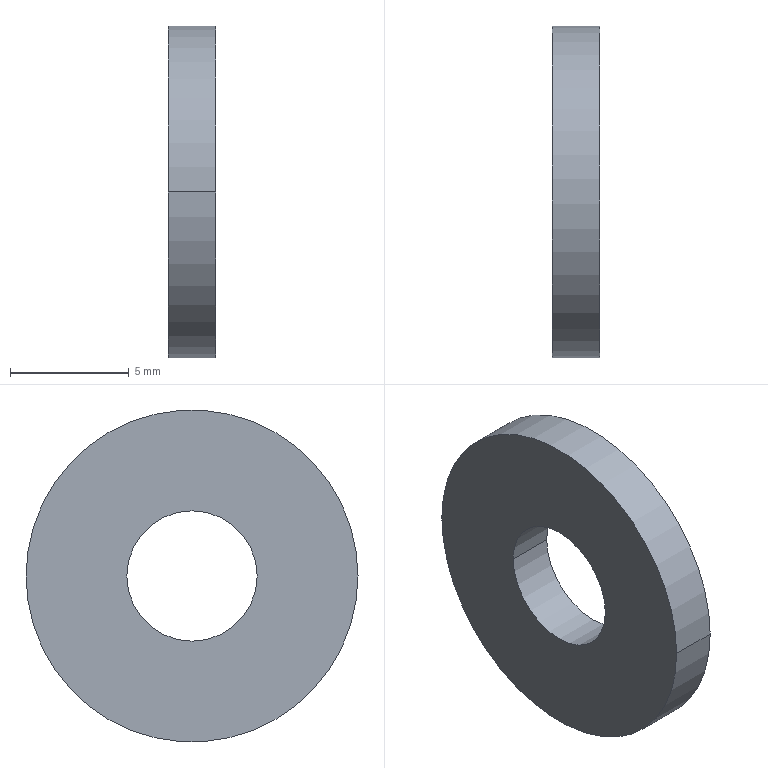Component | SolidWorks | 09HHHHHH6-1 | 1 solid | 6 faces | box 2 x 14 x 14 mm | volume 260 mm3 | cylinder 4 | plane 2 | commonest cylinder face diameters 5.5 x2 14 x2
build123d program:
from build123d import *

# Parameters (mm, degrees)
SKETCH1_R           = 7
SKETCH1_R_2         = 2.75
BOSS_EXTRUDE1_DEPTH = 2


with BuildPart() as part:
    # Sketch1 → Boss-Extrude1 (new body)
    with BuildSketch(Plane.XY):
        with Locations((302.287, -36.6)):
            Circle(SKETCH1_R)
        with Locations((302.287, -36.6)):
            Circle(SKETCH1_R_2, mode=Mode.SUBTRACT)
    extrude(amount=BOSS_EXTRUDE1_DEPTH)


solid = part.part

# Placed as in the assembly
solid = solid.moved(Location((-649.859, -249.783, 272.031), (0, 90, 0)))
STEP:
#1=COLOUR_RGB('',0.7922,0.8196,0.9333);
#2=FILL_AREA_STYLE_COLOUR('',#1);
#3=FILL_AREA_STYLE('',(#2));
#4=SURFACE_STYLE_FILL_AREA(#3);
#5=SURFACE_SIDE_STYLE('',(#4));
#6=SURFACE_STYLE_USAGE(.BOTH.,#5);
#7=PRESENTATION_STYLE_ASSIGNMENT((#6));
#8=CARTESIAN_POINT('',(-25.585,-11.167,-1.191));
#9=VERTEX_POINT('',#8);
#10=CARTESIAN_POINT('',(-25.585,-11.383,-1.191));
#11=VERTEX_POINT('',#10);
#12=CARTESIAN_POINT('',(-25.585,-11.275,-1.191));
#13=DIRECTION('',(-1.,0.,0.));
#14=DIRECTION('',(0.,-1.,0.));
#15=AXIS2_PLACEMENT_3D('',#12,#13,#14);
#16=CIRCLE('',#15,0.1083);
#17=EDGE_CURVE('',#9,#11,#16,.T.);
#18=ORIENTED_EDGE('',*,*,#17,.T.);
#19=CARTESIAN_POINT('',(-25.506,-11.383,-1.191));
#20=VERTEX_POINT('',#19);
#21=CARTESIAN_POINT('',(-25.585,-11.383,-1.191));
#22=DIRECTION('',(1.,0.,0.));
#23=VECTOR('',#22,39.37);
#24=LINE('',#21,#23);
#25=EDGE_CURVE('',#11,#20,#24,.T.);
#26=ORIENTED_EDGE('',*,*,#25,.T.);
#27=CARTESIAN_POINT('',(-25.506,-11.167,-1.191));
#28=VERTEX_POINT('',#27);
#29=CARTESIAN_POINT('',(-25.506,-11.275,-1.191));
#30=DIRECTION('',(-1.,0.,0.));
#31=DIRECTION('',(0.,-1.,0.));
#32=AXIS2_PLACEMENT_3D('',#29,#30,#31);
#33=CIRCLE('',#32,0.1083);
#34=EDGE_CURVE('',#28,#20,#33,.T.);
#35=ORIENTED_EDGE('',*,*,#34,.F.);
#36=CARTESIAN_POINT('',(-25.585,-11.167,-1.191));
#37=DIRECTION('',(1.,0.,0.));
#38=VECTOR('',#37,39.37);
#39=LINE('',#36,#38);
#40=EDGE_CURVE('',#9,#28,#39,.T.);
#41=ORIENTED_EDGE('',*,*,#40,.F.);
#42=EDGE_LOOP('',(#18,#26,#35,#41));
#43=FACE_OUTER_BOUND('',#42,.T.);
#44=CARTESIAN_POINT('',(-25.585,-11.275,-1.191));
#45=DIRECTION('',(1.,0.,0.));
#46=DIRECTION('',(0.,1.,0.));
#47=AXIS2_PLACEMENT_3D('',#44,#45,#46);
#48=CYLINDRICAL_SURFACE('',#47,0.1083);
#49=ADVANCED_FACE('',(#43),#48,.F.);
#50=CARTESIAN_POINT('',(-25.585,-11.551,-1.191));
#51=VERTEX_POINT('',#50);
#52=CARTESIAN_POINT('',(-25.585,-10.999,-1.191));
#53=VERTEX_POINT('',#52);
#54=CARTESIAN_POINT('',(-25.585,-11.275,-1.191));
#55=DIRECTION('',(-1.,0.,0.));
#56=DIRECTION('',(0.,-1.,0.));
#57=AXIS2_PLACEMENT_3D('',#54,#55,#56);
#58=CIRCLE('',#57,0.2756);
#59=EDGE_CURVE('',#51,#53,#58,.T.);
#60=ORIENTED_EDGE('',*,*,#59,.F.);
#61=CARTESIAN_POINT('',(-25.506,-11.551,-1.191));
#62=VERTEX_POINT('',#61);
#63=CARTESIAN_POINT('',(-25.585,-11.551,-1.191));
#64=DIRECTION('',(1.,0.,0.));
#65=VECTOR('',#64,39.37);
#66=LINE('',#63,#65);
#67=EDGE_CURVE('',#51,#62,#66,.T.);
#68=ORIENTED_EDGE('',*,*,#67,.T.);
#69=CARTESIAN_POINT('',(-25.506,-10.999,-1.191));
#70=VERTEX_POINT('',#69);
#71=CARTESIAN_POINT('',(-25.506,-11.275,-1.191));
#72=DIRECTION('',(-1.,0.,0.));
#73=DIRECTION('',(0.,-1.,0.));
#74=AXIS2_PLACEMENT_3D('',#71,#72,#73);
#75=CIRCLE('',#74,0.2756);
#76=EDGE_CURVE('',#62,#70,#75,.T.);
#77=ORIENTED_EDGE('',*,*,#76,.T.);
#78=CARTESIAN_POINT('',(-25.585,-10.999,-1.191));
#79=DIRECTION('',(1.,0.,0.));
#80=VECTOR('',#79,39.37);
#81=LINE('',#78,#80);
#82=EDGE_CURVE('',#53,#70,#81,.T.);
#83=ORIENTED_EDGE('',*,*,#82,.F.);
#84=EDGE_LOOP('',(#60,#68,#77,#83));
#85=FACE_OUTER_BOUND('',#84,.T.);
#86=CARTESIAN_POINT('',(-25.585,-11.275,-1.191));
#87=DIRECTION('',(1.,0.,0.));
#88=DIRECTION('',(0.,1.,0.));
#89=AXIS2_PLACEMENT_3D('',#86,#87,#88);
#90=CYLINDRICAL_SURFACE('',#89,0.2756);
#91=ADVANCED_FACE('',(#85),#90,.T.);
#92=CARTESIAN_POINT('',(-25.585,-11.275,-1.191));
#93=DIRECTION('',(-1.,0.,0.));
#94=DIRECTION('',(0.,-1.,0.));
#95=AXIS2_PLACEMENT_3D('',#92,#93,#94);
#96=CIRCLE('',#95,0.2756);
#97=EDGE_CURVE('',#53,#51,#96,.T.);
#98=ORIENTED_EDGE('',*,*,#97,.T.);
#99=ORIENTED_EDGE('',*,*,#59,.T.);
#100=EDGE_LOOP('',(#98,#99));
#101=FACE_OUTER_BOUND('',#100,.T.);
#102=ORIENTED_EDGE('',*,*,#17,.F.);
#103=CARTESIAN_POINT('',(-25.585,-11.275,-1.191));
#104=DIRECTION('',(-1.,0.,0.));
#105=DIRECTION('',(0.,-1.,0.));
#106=AXIS2_PLACEMENT_3D('',#103,#104,#105);
#107=CIRCLE('',#106,0.1083);
#108=EDGE_CURVE('',#11,#9,#107,.T.);
#109=ORIENTED_EDGE('',*,*,#108,.F.);
#110=EDGE_LOOP('',(#102,#109));
#111=FACE_BOUND('',#110,.T.);
#112=CARTESIAN_POINT('',(-25.585,-11.275,-1.191));
#113=DIRECTION('',(-1.,0.,0.));
#114=DIRECTION('',(0.,-1.,0.));
#115=AXIS2_PLACEMENT_3D('',#112,#113,#114);
#116=PLANE('',#115);
#117=ADVANCED_FACE('',(#101,#111),#116,.T.);
#118=CARTESIAN_POINT('',(-25.506,-11.275,-1.191));
#119=DIRECTION('',(-1.,0.,0.));
#120=DIRECTION('',(0.,-1.,0.));
#121=AXIS2_PLACEMENT_3D('',#118,#119,#120);
#122=CIRCLE('',#121,0.2756);
#123=EDGE_CURVE('',#70,#62,#122,.T.);
#124=ORIENTED_EDGE('',*,*,#123,.F.);
#125=ORIENTED_EDGE('',*,*,#76,.F.);
#126=EDGE_LOOP('',(#124,#125));
#127=FACE_OUTER_BOUND('',#126,.T.);
#128=ORIENTED_EDGE('',*,*,#34,.T.);
#129=CARTESIAN_POINT('',(-25.506,-11.275,-1.191));
#130=DIRECTION('',(-1.,0.,0.));
#131=DIRECTION('',(0.,-1.,0.));
#132=AXIS2_PLACEMENT_3D('',#129,#130,#131);
#133=CIRCLE('',#132,0.1083);
#134=EDGE_CURVE('',#20,#28,#133,.T.);
#135=ORIENTED_EDGE('',*,*,#134,.T.);
#136=EDGE_LOOP('',(#128,#135));
#137=FACE_BOUND('',#136,.T.);
#138=CARTESIAN_POINT('',(-25.506,-11.275,-1.191));
#139=DIRECTION('',(-1.,0.,0.));
#140=DIRECTION('',(0.,-1.,0.));
#141=AXIS2_PLACEMENT_3D('',#138,#139,#140);
#142=PLANE('',#141);
#143=ADVANCED_FACE('',(#127,#137),#142,.F.);
#144=ORIENTED_EDGE('',*,*,#67,.F.);
#145=ORIENTED_EDGE('',*,*,#97,.F.);
#146=ORIENTED_EDGE('',*,*,#82,.T.);
#147=ORIENTED_EDGE('',*,*,#123,.T.);
#148=EDGE_LOOP('',(#144,#145,#146,#147));
#149=FACE_OUTER_BOUND('',#148,.T.);
#150=CARTESIAN_POINT('',(-25.585,-11.275,-1.191));
#151=DIRECTION('',(1.,0.,0.));
#152=DIRECTION('',(0.,1.,0.));
#153=AXIS2_PLACEMENT_3D('',#150,#151,#152);
#154=CYLINDRICAL_SURFACE('',#153,0.2756);
#155=ADVANCED_FACE('',(#149),#154,.T.);
#156=ORIENTED_EDGE('',*,*,#25,.F.);
#157=ORIENTED_EDGE('',*,*,#108,.T.);
#158=ORIENTED_EDGE('',*,*,#40,.T.);
#159=ORIENTED_EDGE('',*,*,#134,.F.);
#160=EDGE_LOOP('',(#156,#157,#158,#159));
#161=FACE_OUTER_BOUND('',#160,.T.);
#162=CARTESIAN_POINT('',(-25.585,-11.275,-1.191));
#163=DIRECTION('',(1.,0.,0.));
#164=DIRECTION('',(0.,1.,0.));
#165=AXIS2_PLACEMENT_3D('',#162,#163,#164);
#166=CYLINDRICAL_SURFACE('',#165,0.1083);
#167=ADVANCED_FACE('',(#161),#166,.F.);
#168=CLOSED_SHELL('',(#49,#91,#117,#143,#155,#167));
#169=MANIFOLD_SOLID_BREP('',#168);
#170=STYLED_ITEM('',(#7),#169);
#171=PRESENTATION_LAYER_ASSIGNMENT('','',(#170));
#172=(LENGTH_UNIT()NAMED_UNIT(*)SI_UNIT($,.METRE.));
#173=LENGTH_MEASURE_WITH_UNIT(LENGTH_MEASURE(0.0254),#172);
#174=DIMENSIONAL_EXPONENTS(1.,0.,0.,0.,0.,0.,0.);
#175=(CONVERSION_BASED_UNIT('',#173)LENGTH_UNIT()NAMED_UNIT(#174));
#176=UNCERTAINTY_MEASURE_WITH_UNIT(LENGTH_MEASURE(0.00001),#175,'','');
#177=(NAMED_UNIT(*)PLANE_ANGLE_UNIT()SI_UNIT($,.RADIAN.));
#178=(NAMED_UNIT(*)SI_UNIT($,.STERADIAN.)SOLID_ANGLE_UNIT());
#179=(GEOMETRIC_REPRESENTATION_CONTEXT(3)GLOBAL_UNCERTAINTY_ASSIGNED_CONTEXT((#176))GLOBAL_UNIT_ASSIGNED_CONTEXT((#175,#177,#178))REPRESENTATION_CONTEXT('',''));
#180=MECHANICAL_DESIGN_GEOMETRIC_PRESENTATION_REPRESENTATION('',(#170),#179);
#181=CARTESIAN_POINT('',(0.,0.,0.));
#182=DIRECTION('',(0.,0.,1.));
#183=DIRECTION('',(1.,0.,0.));
#184=AXIS2_PLACEMENT_3D('',#181,#182,#183);
#185=(LENGTH_UNIT()NAMED_UNIT(*)SI_UNIT($,.METRE.));
#186=LENGTH_MEASURE_WITH_UNIT(LENGTH_MEASURE(0.0254),#185);
#187=DIMENSIONAL_EXPONENTS(1.,0.,0.,0.,0.,0.,0.);
#188=(CONVERSION_BASED_UNIT('',#186)LENGTH_UNIT()NAMED_UNIT(#187));
#189=UNCERTAINTY_MEASURE_WITH_UNIT(LENGTH_MEASURE(0.00001),#188,'','');
#190=(NAMED_UNIT(*)PLANE_ANGLE_UNIT()SI_UNIT($,.RADIAN.));
#191=(NAMED_UNIT(*)SI_UNIT($,.STERADIAN.)SOLID_ANGLE_UNIT());
#192=(GEOMETRIC_REPRESENTATION_CONTEXT(3)GLOBAL_UNCERTAINTY_ASSIGNED_CONTEXT((#189))GLOBAL_UNIT_ASSIGNED_CONTEXT((#188,#190,#191))REPRESENTATION_CONTEXT('',''));
#193=ADVANCED_BREP_SHAPE_REPRESENTATION('',(#169,#184),#192);